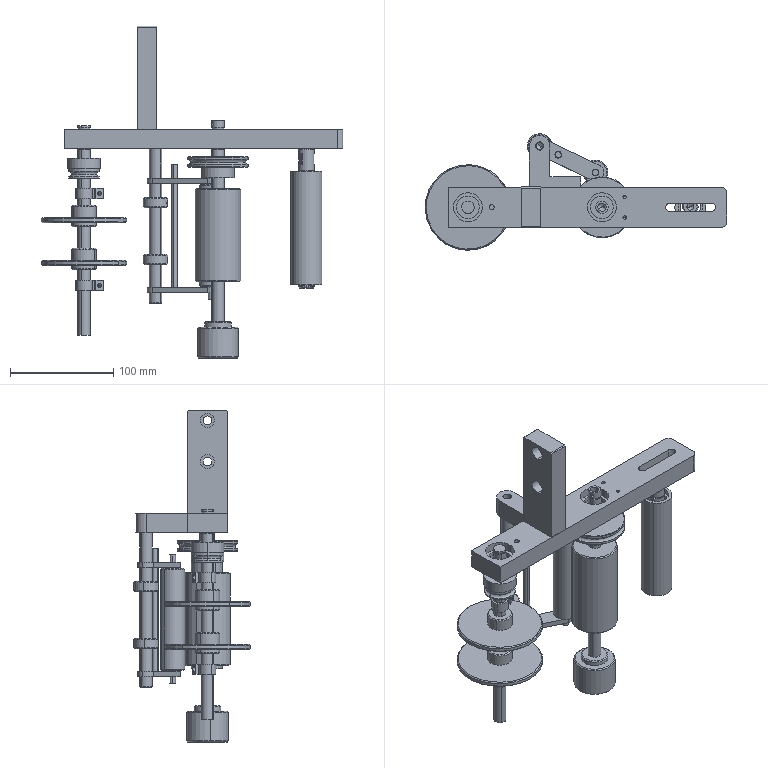Assembly | SolidWorks | mm | 23 component files | 23 solids | 441 faces | box 292.5 x 113 x 322.1 mm | volume 714073 mm3 | cylinder 230 | plane 127 | cone 76 | torus 8 | commonest cylinder face diameters 12 x38 24 x18 16 x14 4.2 x12 6.5 x10 28 x8 13.5 x8 8.5 x8
Bill of materials:
TAR-01-28PaperSupportRollerAxis | 1 |  | Long solid cylindrical rod. One end has a short stepped section with a flat milled on the side, and an axial blind hole with a cone-shaped bottom. Both ends have small chamfers.
TAR-01-39Roller | 1 |  | Plain thin-walled cylindrical tube with a through bore that runs the full length. Ends are square.
TAR-02-017RightSupportPlate | 1 |  | Rectangular block with two round through holes in a line along its long axis, passing through the thickness. Some edges have small chamfers.
TAR-02-019PaperCollectionMotorPlate | 1 |  | Long flat rectangular bar with rounded corners at one end. It has several through features: two large stepped (counterbored) holes, one small single hole, a pair of medium holes, a pair of very small holes, and one elongated slot near the rounded end.
TAR-02-022PaperPressWheelSeat | 1 |  | L-shaped bracket made from thick plate. One arm ends in a rounded end with a through hole running in the thickness direction. The other arm has two through holes in its side face, at right angles to the first hole.
TAR-02-023KnurledPaperPressWheel | 1 |  | Thick-walled cylindrical tube or sleeve with a through bore and chamfered outer edges at both ends.
TAR-02-024PaperPressWheelAxis | 1 |  | Solid stepped shaft: a long central section of larger diameter, with a shorter, smaller-diameter section at each end.
TAR-02-025PaperFeedMotorAxis | 1 |  | Long slender cylindrical rod with an axial blind hole at one end and two narrow circumferential grooves or edge lines near that same end.
TAR-02-026SmallPulleyAxis | 1 |  | Long slender solid cylindrical rod with two narrow circumferential grooves near one end and a slight chamfer at that end.
TAR-02-030CoarseKnurledHandwheel | 1 |  | Short stepped cylinder: a large-diameter main body with a smaller concentric boss on one face, and a central through hole. The outer edges are chamfered.
TAR-02-031LargePulley | 1 |  | Disc-shaped wheel with a semicircular groove around its rim between two flanges, a central through bore, and a cylindrical hub projecting from one face. The hub has one radial hole.
TAR-02-032SmallPulley | 1 |  | Cylindrical body with a central through bore. A larger-diameter section has a single radial hole. Below it is a slightly smaller section that carries a semicircular groove around its circumference, ending in a flange.
TAR-02-033PaperStopWheel | 2 |  | Thin circular disc flange with a short cylindrical hub at its center. The hub sticks out on both faces, and a through bore runs along the axis.
TAR-02-034PaperRollWheel | 1 |  | Thick-walled cylindrical sleeve with a small axial through bore.
TAR-02-035TieRod | 1 |  | Long, slender, solid round rod or pin with flat ends.
TAR-02-036SpringFixingSleeve | 2 |  | Ring-shaped collar with a large central bore, chamfered outer edges, one radial hole through the side wall and one small offset axial hole in one face.
TAR-02-037FixingPlate | 2 |  | Flat bar link of constant thickness with rounded ends and three through holes in a line: a large hole at one end and two smaller holes along the bar.
TAR-02-038ShaftClampBlock | 2 |  | Split ring clamp body: a cylindrical ring with a radial slot that opens between two parallel rectangular lugs, a cross hole running through both lugs, and rounded relief notches at the root of the slot.
TAR-02-081PaperRollAxis | 1 |  | Long, slender cylindrical tube or rod with a concentric axial hole visible at one end.
Mates:
1. concentric | TAR-02-019PaperCollectionMotorPlate-1 face at (-115.391, 9.288, -1.5) dir (0, 0, -1) r 14 | TAR-02-026SmallPulleyAxis-1 face at (-115.391, 9.288, -190.4) dir (0, 0, 1) r 6
2. coincident | TAR-02-019PaperCollectionMotorPlate-1 face at (130.609, 23.788, -9.5) dir (0, 0, -1) | TAR-02-026SmallPulleyAxis-1 face at (-115.391, 9.288, -9.5) dir (0, 0, -1)
3. concentric | TAR-02-026SmallPulleyAxis-1 face at (-115.391, 9.288, -190.4) dir (0, 0, 1) r 6 | TAR-02-033PaperStopWheel-1 face at (-115.391, 9.288, -163.4) dir (0, 0, 1) r 6
4. concentric | TAR-02-026SmallPulleyAxis-1 face at (-115.391, 9.288, -190.4) dir (0, 0, 1) r 6 | TAR-02-038ShaftClampBlock-2 face at (-115.391, 9.288, -47.94) dir (0, 0, -1) r 6
5. concentric | TAR-02-026SmallPulleyAxis-1 face at (-115.391, 9.288, -190.4) dir (0, 0, 1) r 6 | TAR-02-033PaperStopWheel-2 face at (-115.391, 9.288, -204.899) dir (0, 0, 1) r 6
6. concentric | TAR-02-026SmallPulleyAxis-1 face at (-115.391, 9.288, -190.4) dir (0, 0, 1) r 6 | TAR-02-038ShaftClampBlock-1 face at (-115.391, 9.288, -137.058) dir (0, 0, -1) r 6
7. concentric | TAR-02-026SmallPulleyAxis-1 face at (-115.391, 9.288, -190.4) dir (0, 0, 1) r 6 | TAR-02-032SmallPulley-1 face at (-115.391, 9.288, 60.377) dir (0, 0, -1) r 6
8. coincident | TAR-02-019PaperCollectionMotorPlate-1 face at (130.609, 23.788, 9.5) dir (0, 0, 1) | TAR-02-017RightSupportPlate-1 face at (-63.891, 28.788, 9.5) dir (0, 0, -1)
9. concentric | TAR-02-019PaperCollectionMotorPlate-1 face at (-54.391, -0.7123, -9.5) dir (0, 0, -1) r 6.75 | TAR-02-017RightSupportPlate-1 face at (-54.391, -0.7123, 9.5) dir (0, 0, -1) r 3.4
10. concentric | TAR-02-019PaperCollectionMotorPlate-1 face at (-54.391, 19.288, -9.5) dir (0, 0, -1) r 4.25 | TAR-02-017RightSupportPlate-1 face at (-54.391, 19.288, 9.5) dir (0, 0, -1) r 3.4
11. coincident | TAR-02-019PaperCollectionMotorPlate-1 face at (130.609, 28.788, 9.5) dir (0, 1, 0) | TAR-02-022PaperPressWheelSeat-1 face at (-55.891, 28.788, 9.5) dir (0, -1, 0)
12. concentric | TAR-02-081PaperRollAxis-1 face at (-45.891, 68.788, 0.5) dir (0, 0, -1) r 6 | TAR-02-037FixingPlate-1 face at (-45.891, 68.788, -38.165) dir (0, 0, -1) r 6
13. concentric | TAR-02-081PaperRollAxis-1 face at (-45.891, 68.788, 0.5) dir (0, 0, -1) r 6 | TAR-02-037FixingPlate-2 face at (-45.891, 68.788, -144.165) dir (0, 0, -1) r 6
14. coincident | TAR-02-037FixingPlate-1 face at (-49.316, 61.558, -38.165) dir (-0.4281, -0.9037, 0) | TAR-02-037FixingPlate-2 face at (-49.316, 61.558, -144.165) dir (-0.4281, -0.9037, 0)
15. concentric | TAR-02-037FixingPlate-2 face at (8.333, 43.101, -144.165) dir (0, 0, -1) r 3.25 | TAR-02-023KnurledPaperPressWheel-1 face at (8.333, 43.101, -44.165) dir (0, 0, -1) r 6
16. concentric | TAR-02-037FixingPlate-2 face at (8.333, 43.101, -144.165) dir (0, 0, -1) r 3.25 | TAR-02-024PaperPressWheelAxis-1 face at (8.333, 43.101, -43.165) dir (0, 0, -1) r 4
17. distance | TAR-02-023KnurledPaperPressWheel-1 face at (8.333, 43.101, -143.165) dir (0, 0, -1) | TAR-02-024PaperPressWheelAxis-1 face at (8.333, 43.101, -144.165) dir (0, 0, -1)
18. coincident | TAR-02-037FixingPlate-1 face at (-45.891, 68.788, -43.165) dir (0, 0, -1) | TAR-02-024PaperPressWheelAxis-1 face at (8.333, 43.101, -43.165) dir (0, 0, 1)
19. coincident | TAR-02-037FixingPlate-2 face at (-45.891, 68.788, -144.165) dir (0, 0, 1) | TAR-02-024PaperPressWheelAxis-1 edge at (8.333, 43.101, -144.165) dir (0, 0, 1) r 4
20. concentric | TAR-02-037FixingPlate-2 face at (-27.816, 60.226, -144.165) dir (0, 0, -1) r 3.25 | TAR-02-035TieRod-1 face at (-27.816, 60.226, -24.44) dir (0, 0, -1) r 3
21. concentric | TAR-02-081PaperRollAxis-1 face at (-45.891, 68.788, 0.5) dir (0, 0, -1) r 6 | TAR-02-036SpringFixingSleeve-2 face at (-45.891, 68.788, -112.057) dir (0, 0, -1) r 6.05
22. concentric | TAR-02-081PaperRollAxis-1 face at (-45.891, 68.788, 0.5) dir (0, 0, -1) r 6 | TAR-02-036SpringFixingSleeve-1 face at (-45.891, 68.788, -56.881) dir (0, 0, -1) r 6.05
23. concentric | TAR-02-019PaperCollectionMotorPlate-1 face at (14.609, 9.288, 9.5) dir (0, 0, -1) r 11 | TAR-02-025PaperFeedMotorAxis-1 face at (14.609, 9.288, -9.5) dir (0, 0, 1) r 6
24. coincident | TAR-02-019PaperCollectionMotorPlate-1 face at (130.609, 23.788, -9.5) dir (0, 0, -1) | TAR-02-025PaperFeedMotorAxis-1 face at (14.609, 9.288, -9.5) dir (0, 0, -1)
25. concentric | TAR-02-025PaperFeedMotorAxis-1 face at (14.609, 9.288, -192.6) dir (0, 0, 1) r 6 | TAR-02-034PaperRollWheel-1 face at (14.609, 9.288, -48.439) dir (0, 0, -1) r 6
26. concentric | TAR-02-019PaperCollectionMotorPlate-1 face at (-28.391, 28.788, 0) dir (0, 1, 0) r 2.1 | TAR-02-022PaperPressWheelSeat-1 face at (-28.391, 38.788, 0) dir (0, 1, 0) r 4.5
27. concentric | TAR-02-019PaperCollectionMotorPlate-1 face at (-13.391, 28.788, 0) dir (0, 1, 0) r 2.1 | TAR-02-022PaperPressWheelSeat-1 face at (-13.391, 38.788, 0) dir (0, 1, 0) r 4.5
28. concentric | TAR-02-022PaperPressWheelSeat-1 face at (-45.891, 68.788, 0.5) dir (0, 0, -1) r 6 | TAR-02-081PaperRollAxis-1 face at (-45.891, 68.788, 0.5) dir (0, 0, -1) r 6
29. coincident | TAR-02-022PaperPressWheelSeat-1 face at (-45.891, 68.788, 0.5) dir (0, 0, -1) | TAR-02-081PaperRollAxis-1 face at (-45.891, 68.788, 0.5) dir (0, 0, 1)
30. concentric | TAR-02-025PaperFeedMotorAxis-1 face at (14.609, 9.288, -192.6) dir (0, 0, 1) r 6 | TAR-02-030CoarseKnurledHandwheel-1 edge at (14.609, 9.288, -212.6) dir (0, 0, -1) r 5.5
31. coincident | TAR-02-025PaperFeedMotorAxis-1 face at (14.609, 9.288, -192.6) dir (0, 0, -1) | TAR-02-030CoarseKnurledHandwheel-1 face at (14.609, 9.288, -192.6) dir (0, 0, 1)
32. concentric | TAR-02-025PaperFeedMotorAxis-1 face at (14.609, 9.288, -192.6) dir (0, 0, 1) r 6 | TAR-02-031LargePulley-1 face at (14.609, 9.288, -1.655) dir (0, 0, -1) r 6
33. concentric | TAR-01-28PaperSupportRollerAxis-1 face at (100.319, 9.938, -141.6) dir (0, 0, 1) r 7.5 | TAR-01-39Roller-1 face at (100.319, 9.938, -1022.6) dir (0, 0, 1) r 10
34. coincident | TAR-01-28PaperSupportRollerAxis-1 face at (100.319, 9.938, -31.6) dir (0, 0, 1) | TAR-01-39Roller-1 face at (100.319, 9.938, -31.6) dir (0, 0, 1)
35. coincident | TAR-02-019PaperCollectionMotorPlate-1 face at (130.609, 23.788, -9.5) dir (0, 0, -1) | TAR-01-28PaperSupportRollerAxis-1 face at (100.319, 9.938, -9.5) dir (0, 0, 1)
36. tangent | TAR-02-019PaperCollectionMotorPlate-1 face at (80.609, 13.338, 9.5) dir (0, -1, 0) | TAR-01-28PaperSupportRollerAxis-1 face at (100.319, 9.938, -9.5) dir (0, 0, 1) r 3.4